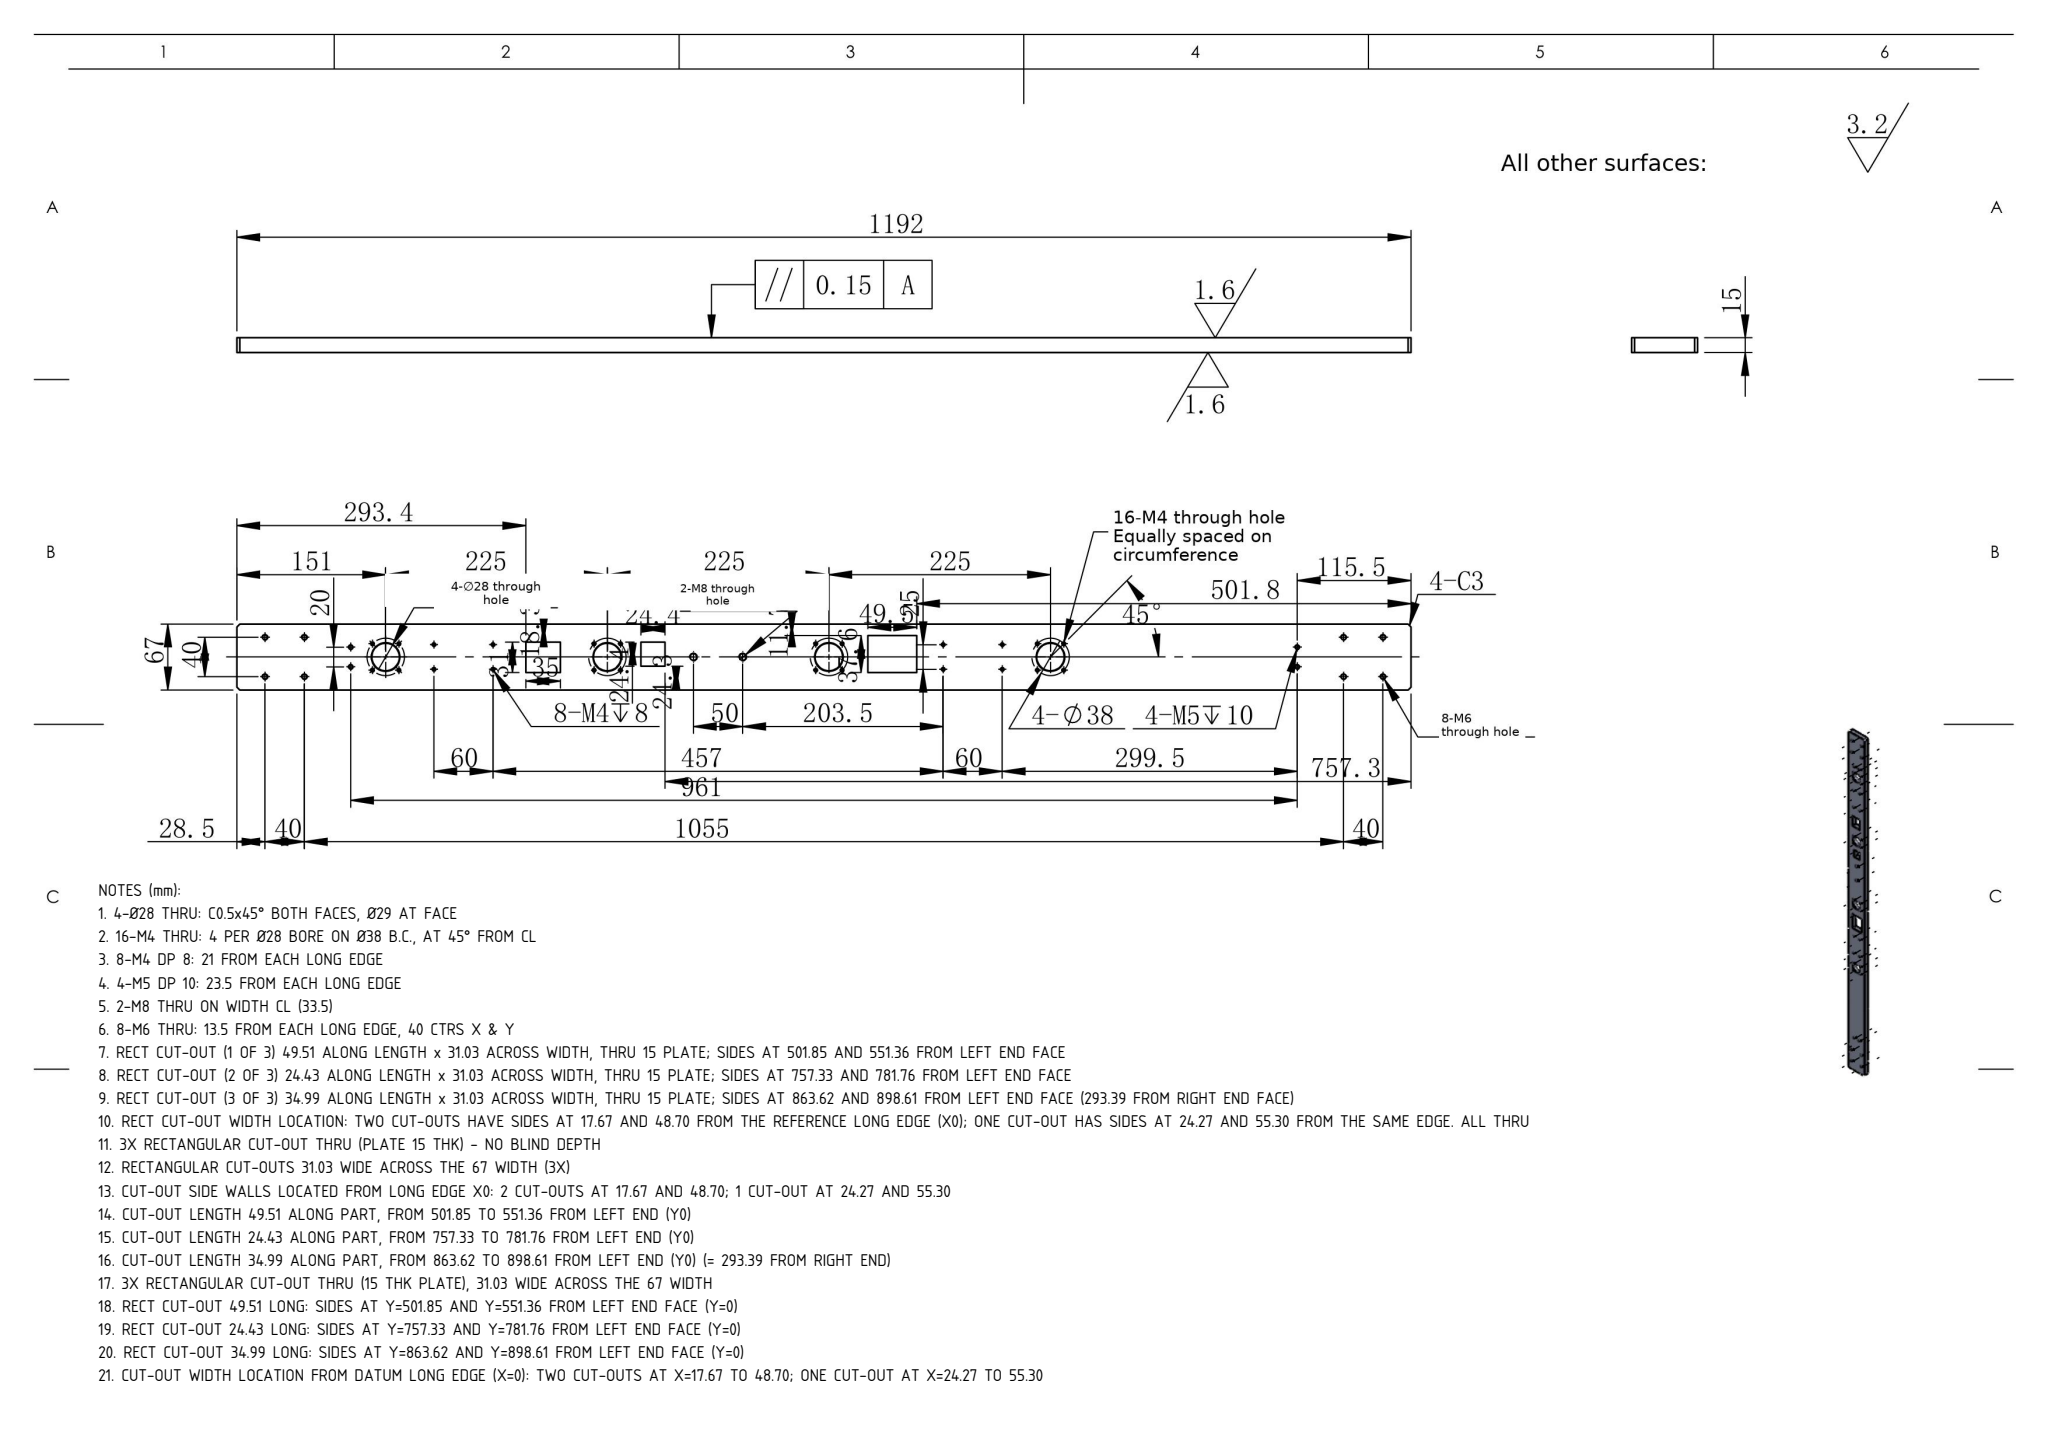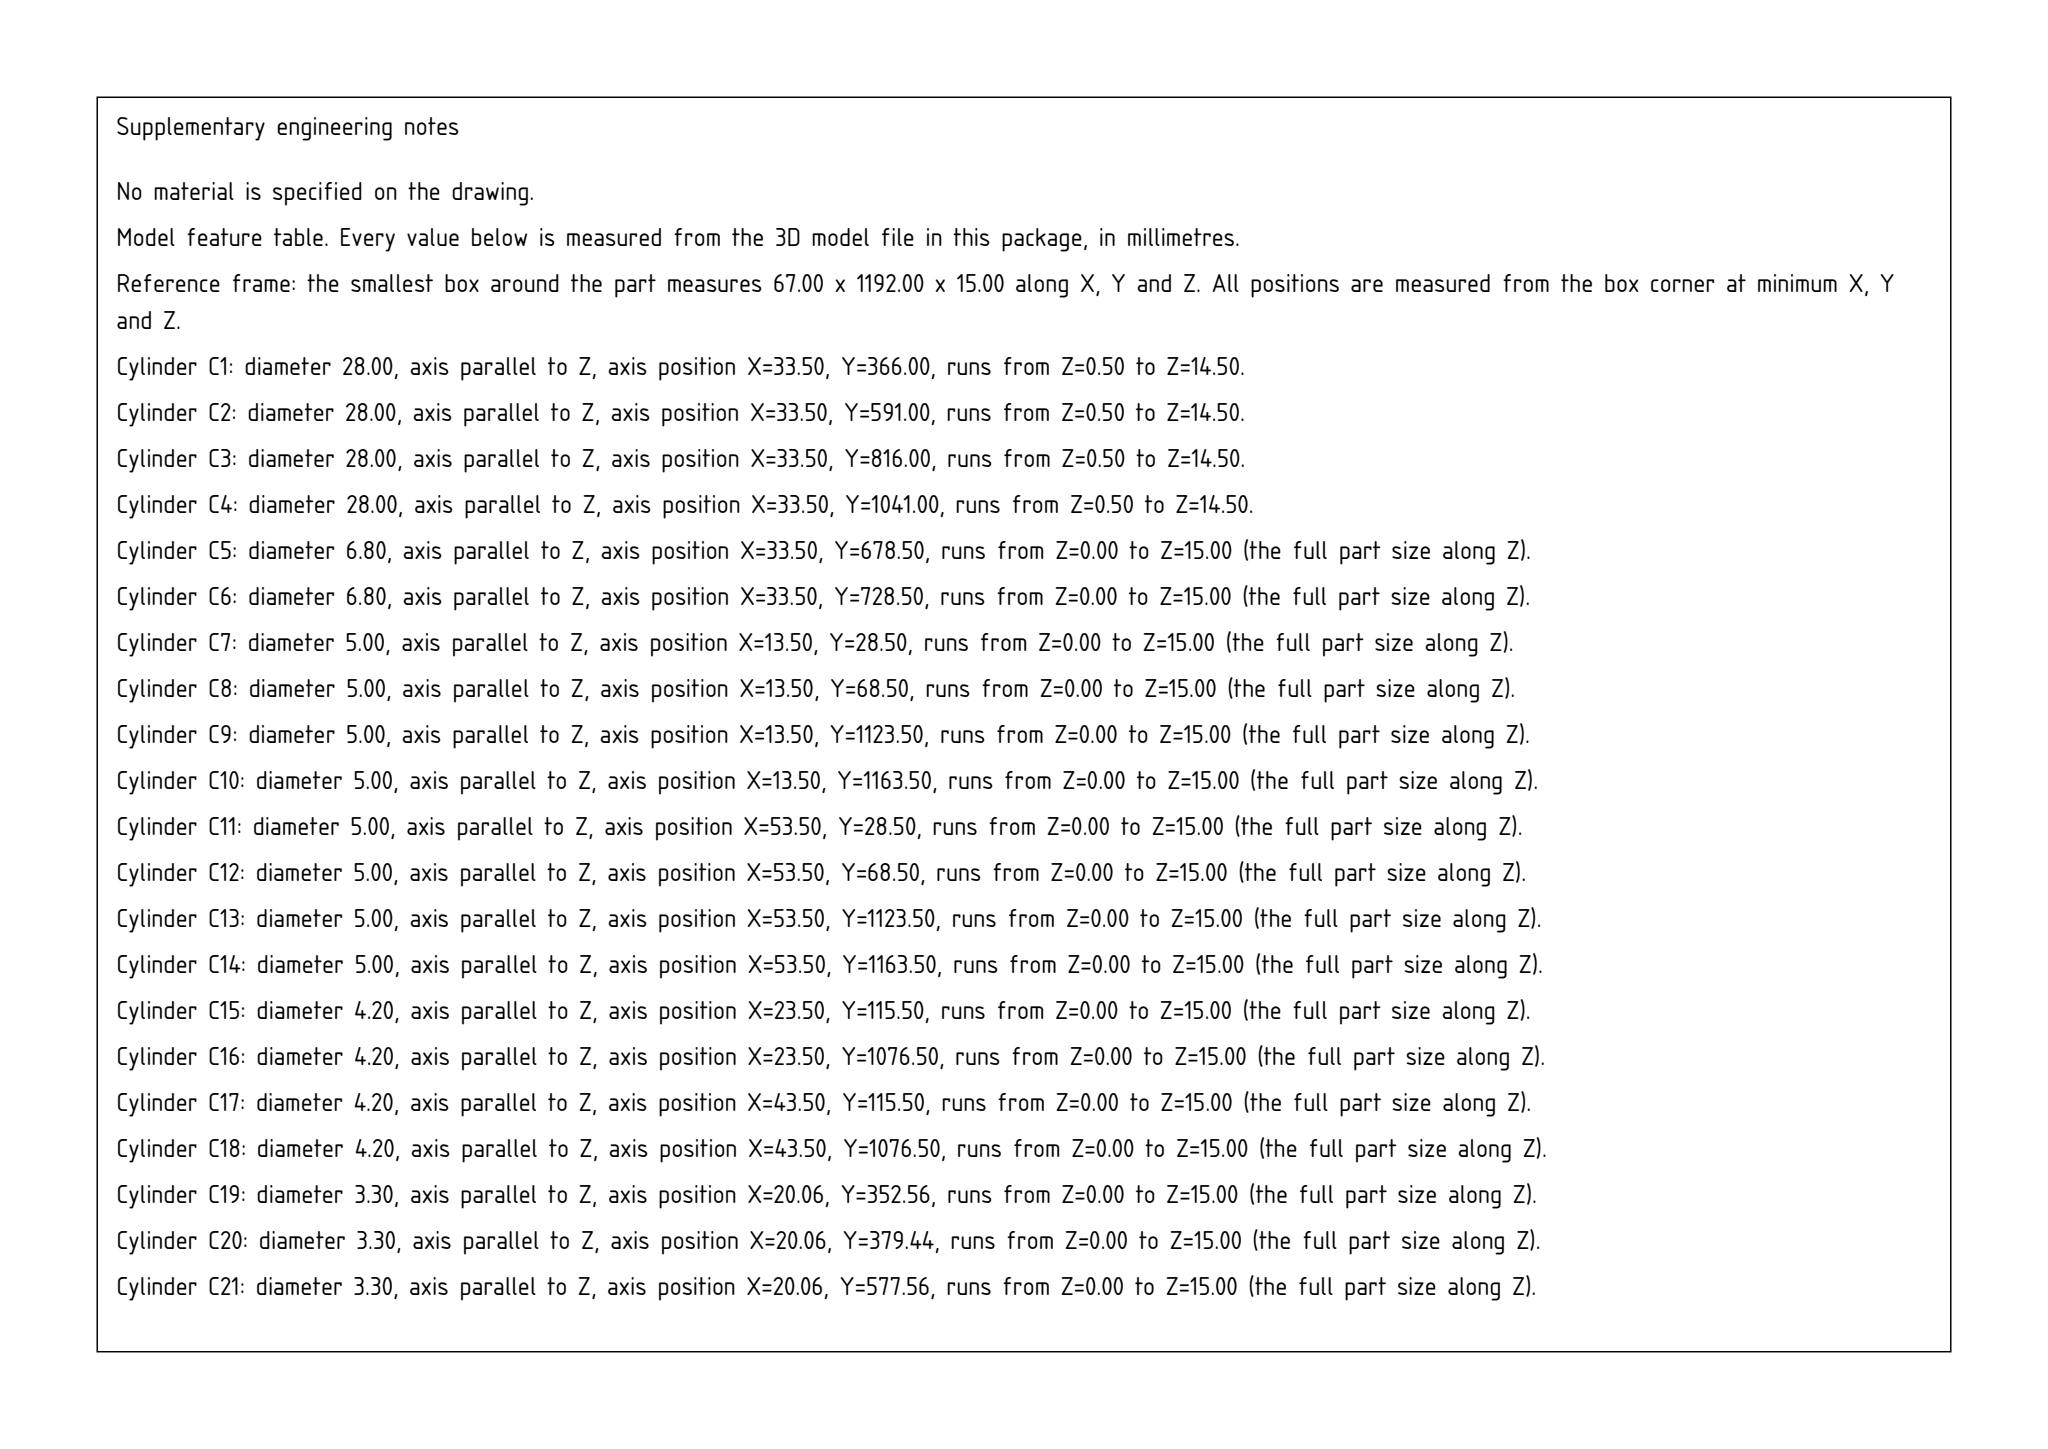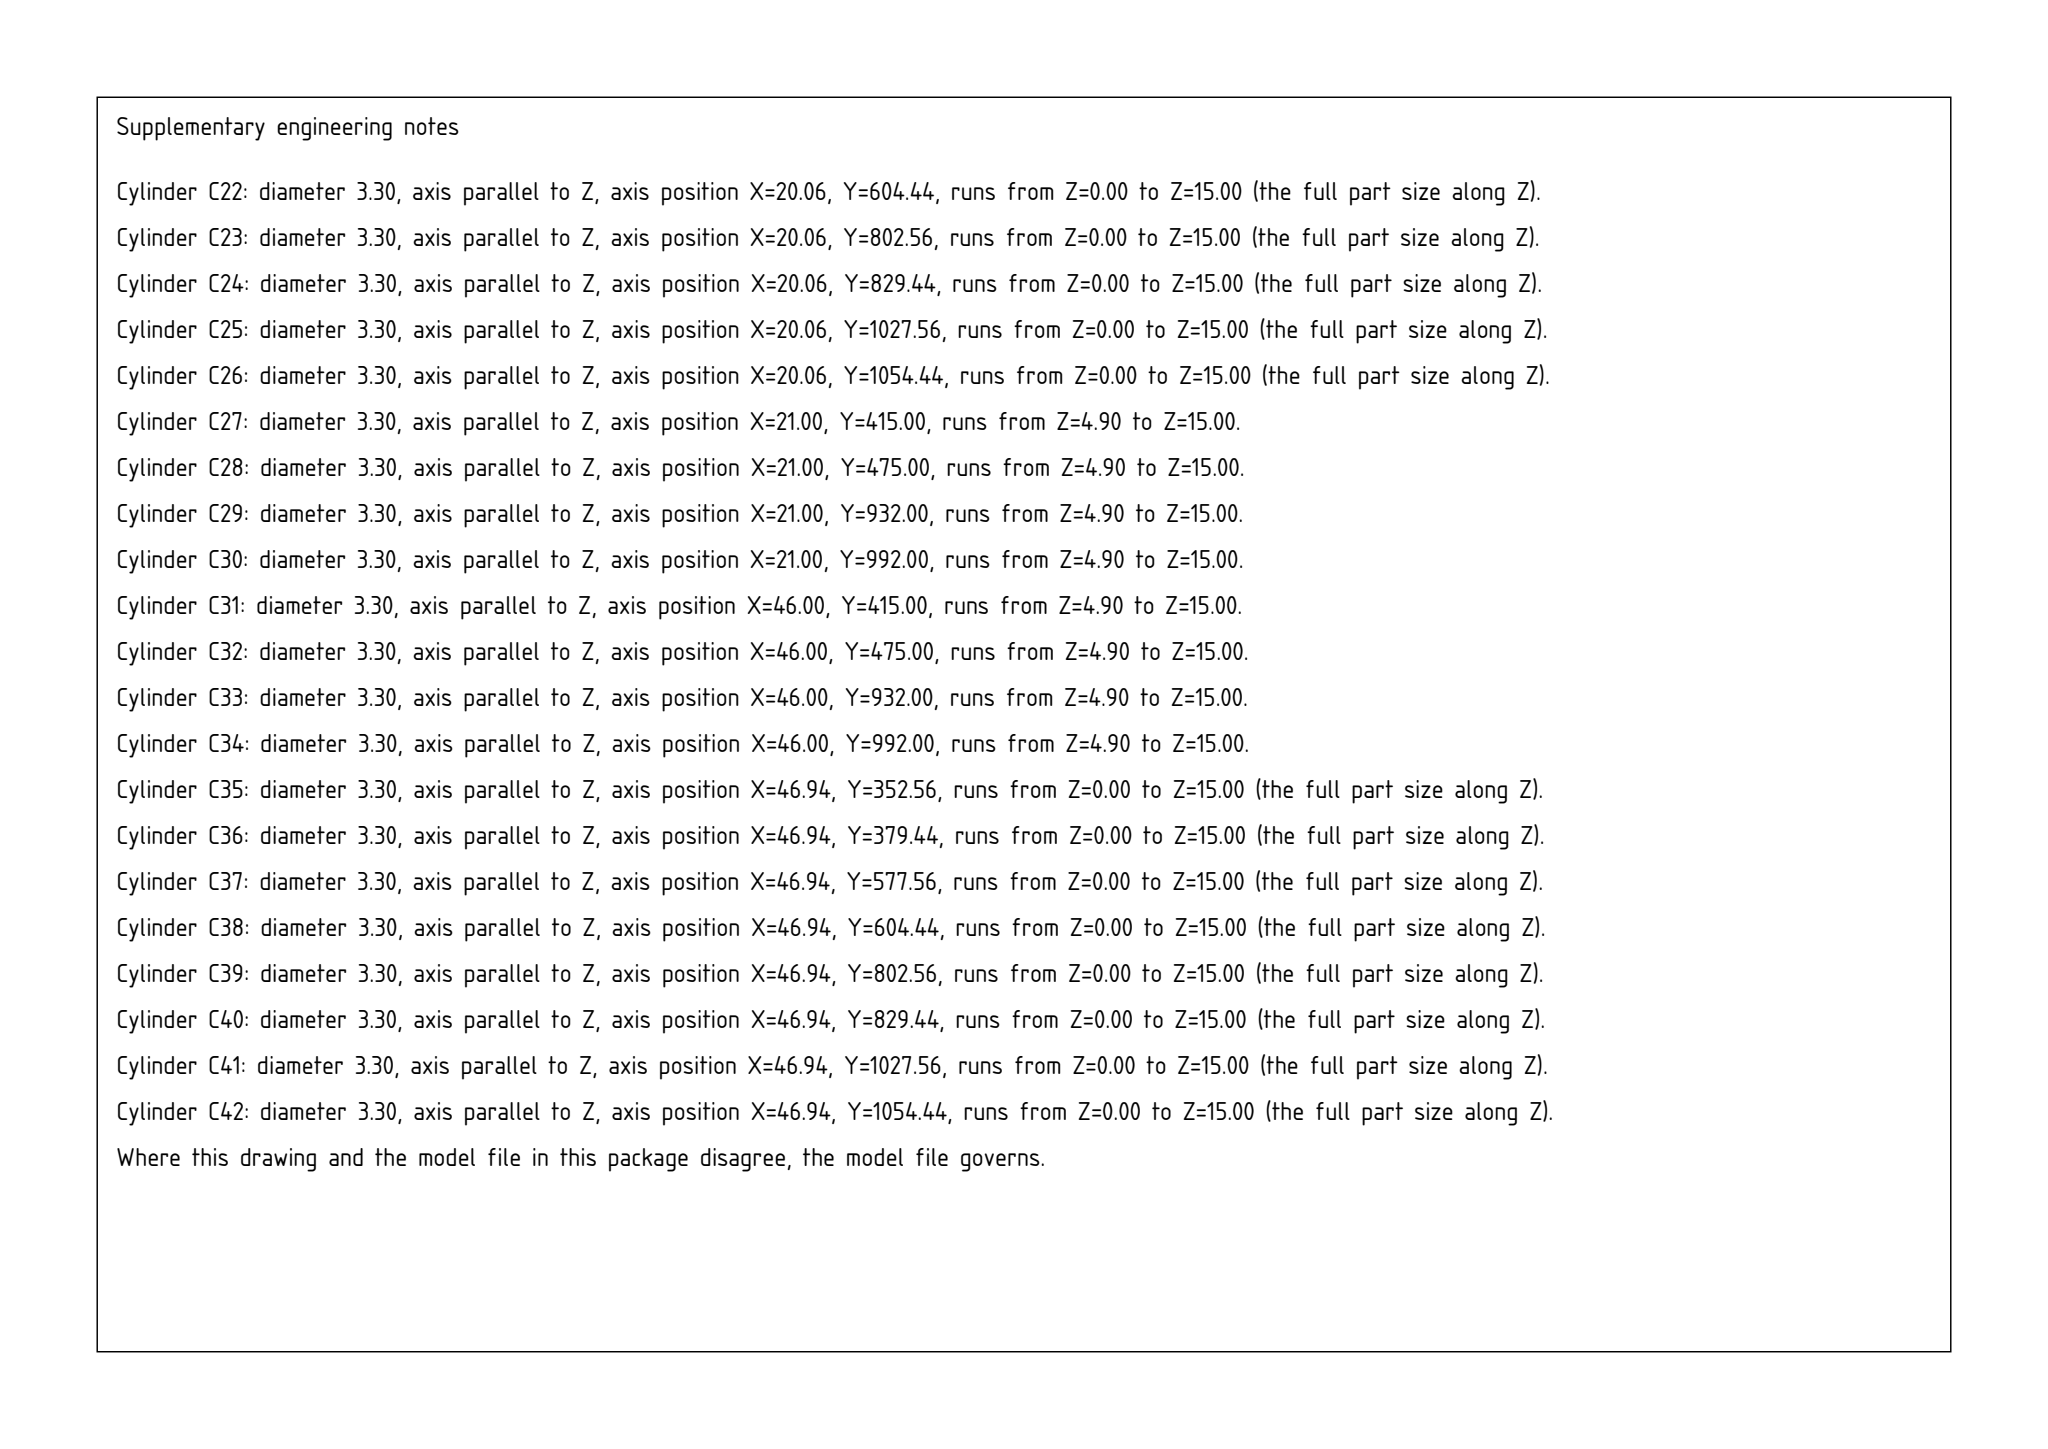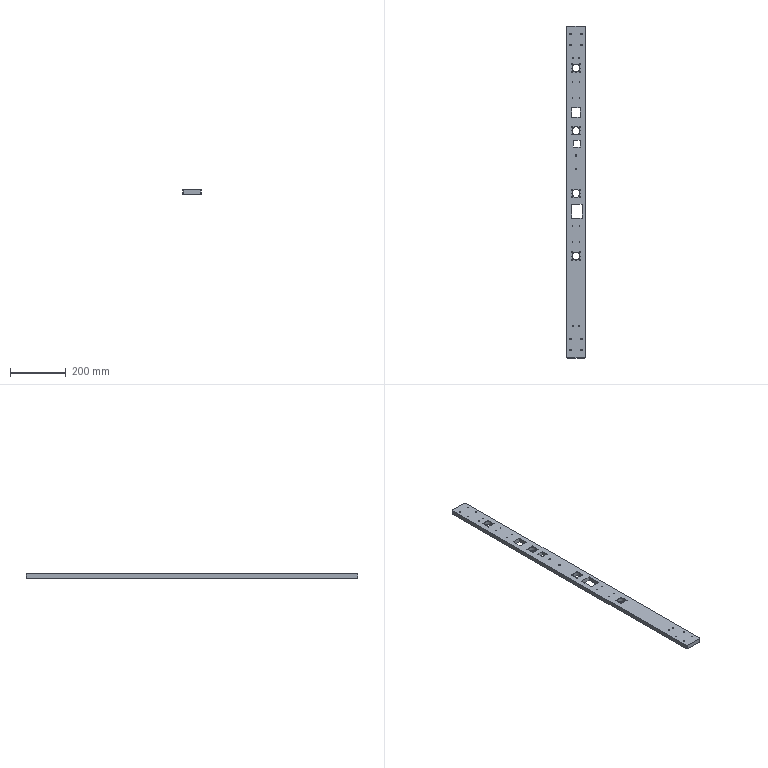Part | SolidWorks | mm | 1 solid | 138 faces | box 67 x 1192 x 15 mm | volume 1100432 mm3 | cylinder 84 | cone 32 | plane 22 | commonest cylinder face diameters 3.3 x48 5 x16 4.2 x8 28 x8 6.8 x4
Drawing notes:
4-Ø28 THRU: C0.5x45° BOTH FACES, Ø29 AT FACE | from the solid: Ø28 cyl L14.0 in 15 thk plate; 90° cones ref dia 28.0 (8) and 29.0 (8)
16-M4 THRU: 4 PER Ø28 BORE ON Ø38 B.C., AT 45° FROM CL | from the solid: Ø3.3 thru at x=20.06/46.94, y=352.56/379.44 etc = ±13.44,±13.44 from bore ctrs (33.5, 366/591/816/1041) -> R19 at 45°
8-M4 DP 8: 21 FROM EACH LONG EDGE | from the solid: Ø3.3 L10.1 at x=21 & 46 (67-46=21)
4-M5 DP 10: 23.5 FROM EACH LONG EDGE | from the solid: Ø4.2 at x=23.5 & 43.5 (67-43.5=23.5)
2-M8 THRU ON WIDTH CL (33.5) | from the solid: Ø6.8 thru at x=33.5 = 67/2 width CL, y=678.5 & 728.5
8-M6 THRU: 13.5 FROM EACH LONG EDGE, 40 CTRS X & Y | from the solid: Ø5.0 thru at x=13.5 & 53.5, y=28.5/68.5 and 1123.5/1163.5; bbox 67 x 1192
RECT CUT-OUT (1 OF 3) 49.51 ALONG LENGTH x 31.03 ACROSS WIDTH, THRU 15 PLATE; SIDES AT 501.85 AND 551.36 FROM LEFT END FACE | from the solid: axis_planes y=501.85 and y=551.36 (49.51 apart); x plane pair spacing 31.03; z planes only 0.0 and 15.0 (no blind floor)
RECT CUT-OUT (2 OF 3) 24.43 ALONG LENGTH x 31.03 ACROSS WIDTH, THRU 15 PLATE; SIDES AT 757.33 AND 781.76 FROM LEFT END FACE | from the solid: axis_planes y=757.33 and y=781.76 (24.43 apart); x plane pair spacing 31.03; z planes only 0.0 and 15.0
RECT CUT-OUT (3 OF 3) 34.99 ALONG LENGTH x 31.03 ACROSS WIDTH, THRU 15 PLATE; SIDES AT 863.62 AND 898.61 FROM LEFT END FACE (293.39 FROM RIGHT END FACE) | from the solid: axis_planes y=863.62 and y=898.61 (34.99 apart); bbox y=1192.0 gives 293.39 to right end; x plane pair spacing 31.03; z planes only 0.0 and 15.0
RECT CUT-OUT WIDTH LOCATION: TWO CUT-OUTS HAVE SIDES AT 17.67 AND 48.70 FROM THE REFERENCE LONG EDGE (X0); ONE CUT-OUT HAS SIDES AT 24.27 AND 55.30 FROM THE SAME EDGE. ALL THRU | from the solid: axis_planes x=17.67 (count 2), x=48.70 (count 2), x=24.27 (count 1), x=55.30 (count 1); bbox x=67.0
3X RECTANGULAR CUT-OUT THRU (PLATE 15 THK) - NO BLIND DEPTH | from the solid: axis_planes z 0.0 and z 15.0 are the only z faces; bbox_xyz z = 15.0, so cut-out walls run full thickness
RECTANGULAR CUT-OUTS 31.03 WIDE ACROSS THE 67 WIDTH (3X) | from the solid: axis_planes x 48.70 - x 17.67 = 31.03 and x 55.30 - x 24.27 = 31.03
CUT-OUT SIDE WALLS LOCATED FROM LONG EDGE X0: 2 CUT-OUTS AT 17.67 AND 48.70; 1 CUT-OUT AT 24.27 AND 55.30 | from the solid: axis_planes x 17.67 count 2, x 48.70 count 2, x 24.27 count 1, x 55.30 count 1
CUT-OUT LENGTH 49.51 ALONG PART, FROM 501.85 TO 551.36 FROM LEFT END (Y0) | from the solid: axis_planes y 501.85 and y 551.36
CUT-OUT LENGTH 24.43 ALONG PART, FROM 757.33 TO 781.76 FROM LEFT END (Y0) | from the solid: axis_planes y 757.33 and y 781.76
CUT-OUT LENGTH 34.99 ALONG PART, FROM 863.62 TO 898.61 FROM LEFT END (Y0) (= 293.39 FROM RIGHT END) | from the solid: axis_planes y 863.62 and y 898.61; bbox y = 1192.0
3X RECTANGULAR CUT-OUT THRU (15 THK PLATE), 31.03 WIDE ACROSS THE 67 WIDTH | from the solid: axis_planes x 17.67 & 48.70 (and 24.27 & 55.30) give 31.03 opening; z planes 0.0 and 15.0 = through thickness
RECT CUT-OUT 49.51 LONG: SIDES AT Y=501.85 AND Y=551.36 FROM LEFT END FACE (Y=0) | from the solid: axis_planes y 501.85 and y 551.36
RECT CUT-OUT 24.43 LONG: SIDES AT Y=757.33 AND Y=781.76 FROM LEFT END FACE (Y=0) | from the solid: axis_planes y 757.33 and y 781.76
RECT CUT-OUT 34.99 LONG: SIDES AT Y=863.62 AND Y=898.61 FROM LEFT END FACE (Y=0) | from the solid: axis_planes y 863.62 and y 898.61
CUT-OUT WIDTH LOCATION FROM DATUM LONG EDGE (X=0): TWO CUT-OUTS AT X=17.67 TO 48.70; ONE CUT-OUT AT X=24.27 TO 55.30 | from the solid: axis_planes x 17.67 (count 2), 48.70 (count 2), 24.27 (count 1), 55.30 (count 1)
build123d program:
from build123d import *

# Parameters (mm, degrees)
SKETCH1_W             = 67
SKETCH1_H             = 1175
BOSS_EXTRUDE1_DEPTH   = 15
M6_TAPPED_HOLE1_D     = 5
SKETCH4_R             = 14
CUT_EXTRUDE1_DEPTH    = 1178.004
M8_TAPPED_HOLE1_D     = 6.8
M8_TAPPED_HOLE1_DEPTH = 19.75
M8_TAPPED_HOLE1_TIP   = 2.043
M4_TAPPED_HOLE1_D     = 3.3
CIRPATTERN1_COUNT     = 4
LPATTERN1_COUNT       = 4
LPATTERN1_PITCH       = 225
LPATTERN1_COPY_1_D    = 3.3
LPATTERN1_COPY_2_D    = 3.3
LPATTERN1_COPY_3_D    = 3.3
LPATTERN1_COPY_4_D    = 3.3
LPATTERN1_COPY_5_D    = 3.3
LPATTERN1_COPY_6_D    = 3.3
LPATTERN1_COPY_7_D    = 3.3
LPATTERN1_COPY_8_D    = 3.3
LPATTERN1_COPY_9_D    = 3.3
CHAMFER2_SIZE         = 0.5
M4_TAPPED_HOLE2_D     = 3.3
M4_TAPPED_HOLE2_DEPTH = 10.1
M4_TAPPED_HOLE2_TIP   = 0.9914
SKETCH11_W            = 67
SKETCH11_H            = 15
BOSS_EXTRUDE2_DEPTH   = 8.5
SKETCH12_W            = 67
SKETCH12_H            = 15
BOSS_EXTRUDE3_DEPTH   = 8.5
CHAMFER3_SIZE         = 3
M5_TAPPED_HOLE1_D     = 4.2
SKETCH15_W            = 31.028
SKETCH15_H            = 34.989
SKETCH15_W_2          = 24.426
SKETCH15_H_2          = 24.426
SKETCH15_W_3          = 37.629
SKETCH15_H_3          = 49.512
CUT_EXTRUDE2_DEPTH    = 104


with BuildPart() as part:
    # Sketch1 → Boss-Extrude1 (new body)
    with BuildSketch(Plane.XY):
        with Locations((33.5, 587.5)):
            Rectangle(SKETCH1_W, SKETCH1_H)
    extrude(amount=BOSS_EXTRUDE1_DEPTH)

    # M6 Tapped Hole1 (through all)
    with Locations(Plane.XY.offset(15)):
        with Locations((13.5, 1155), (53.5, 1155), (53.5, 1115), (13.5, 1115), (13.5, 60), (53.5, 60), (53.5, 20), (13.5, 20)):
            Hole(M6_TAPPED_HOLE1_D / 2)

    # Sketch4 → Cut-Extrude1 (cut, through all)
    with BuildSketch(Plane.XY.offset(15)):
        with Locations((33.5, 1032.5)):
            Circle(SKETCH4_R)
        with Locations(Location((33.5, 357.5, 0), (0, 0, 180))):
            Circle(SKETCH4_R)
        with Locations((33.5, 807.5)):
            Circle(SKETCH4_R)
        with Locations(Location((33.5, 582.5, 0), (0, 0, 180))):
            Circle(SKETCH4_R)
    extrude(amount=-CUT_EXTRUDE1_DEPTH, mode=Mode.SUBTRACT)

    # M8 Tapped Hole1
    with Locations(Plane.XY.offset(15)):
        with Locations((33.5, 720), (33.5, 670)):
            Hole(M8_TAPPED_HOLE1_D / 2, depth=M8_TAPPED_HOLE1_DEPTH)
            with Locations((0, 0, -(M8_TAPPED_HOLE1_DEPTH + M8_TAPPED_HOLE1_TIP / 2))):  # 118° drill point
                Cone(0, M8_TAPPED_HOLE1_D / 2, M8_TAPPED_HOLE1_TIP, mode=Mode.SUBTRACT)

    # M4 Tapped Hole1 (through all)
    with Locations(Plane.XY.offset(15)):
        with Locations((46.935, 1045.935)):
            m4_tapped_hole1 = Hole(M4_TAPPED_HOLE1_D / 2)

    # CirPattern1: M4 Tapped Hole1 ×4 about axis
    cirpattern1_axis = Axis((33.5, 1032.5, 0), (0, 0, 1))
    for i in range(1, CIRPATTERN1_COUNT):
        add(m4_tapped_hole1.rotate(cirpattern1_axis, i * 360 / CIRPATTERN1_COUNT), mode=Mode.SUBTRACT)

    # LPattern1: M4 Tapped Hole1 ×4
    with Locations(*[(0, -i * LPATTERN1_PITCH, 0) for i in range(1, LPATTERN1_COUNT)]):
        add(m4_tapped_hole1, mode=Mode.SUBTRACT)

    # LPattern1 copy 1 (through all)
    with Locations(Plane(origin=(1066, 774, 15), x_dir=(0, 1, 0), z_dir=(0, 0, 1))):
        with Locations((46.935, 1045.935)):
            Hole(LPATTERN1_COPY_1_D / 2)

    # LPattern1 copy 2 (through all)
    with Locations(Plane(origin=(1066, 549, 15), x_dir=(0, 1, 0), z_dir=(0, 0, 1))):
        with Locations((46.935, 1045.935)):
            Hole(LPATTERN1_COPY_2_D / 2)

    # LPattern1 copy 3 (through all)
    with Locations(Plane(origin=(1066, 324, 15), x_dir=(0, 1, 0), z_dir=(0, 0, 1))):
        with Locations((46.935, 1045.935)):
            Hole(LPATTERN1_COPY_3_D / 2)

    # LPattern1 copy 4 (through all)
    with Locations(Plane(origin=(67, 1840, 15), x_dir=(-1, 0, 0), z_dir=(0, 0, 1))):
        with Locations((46.935, 1045.935)):
            Hole(LPATTERN1_COPY_4_D / 2)

    # LPattern1 copy 5 (through all)
    with Locations(Plane(origin=(67, 1615, 15), x_dir=(-1, 0, 0), z_dir=(0, 0, 1))):
        with Locations((46.935, 1045.935)):
            Hole(LPATTERN1_COPY_5_D / 2)

    # LPattern1 copy 6 (through all)
    with Locations(Plane(origin=(67, 1390, 15), x_dir=(-1, 0, 0), z_dir=(0, 0, 1))):
        with Locations((46.935, 1045.935)):
            Hole(LPATTERN1_COPY_6_D / 2)

    # LPattern1 copy 7 (through all)
    with Locations(Plane(origin=(-999, 841, 15), x_dir=(0, -1, 0), z_dir=(0, 0, 1))):
        with Locations((46.935, 1045.935)):
            Hole(LPATTERN1_COPY_7_D / 2)

    # LPattern1 copy 8 (through all)
    with Locations(Plane(origin=(-999, 616, 15), x_dir=(0, -1, 0), z_dir=(0, 0, 1))):
        with Locations((46.935, 1045.935)):
            Hole(LPATTERN1_COPY_8_D / 2)

    # LPattern1 copy 9 (through all)
    with Locations(Plane(origin=(-999, 391, 15), x_dir=(0, -1, 0), z_dir=(0, 0, 1))):
        with Locations((46.935, 1045.935)):
            Hole(LPATTERN1_COPY_9_D / 2)

    # Chamfer2
    chamfer2_edges = [part.edges().sort_by_distance(p)[0] for p in [
        (19.5, 1032.5, 0),
        (19.5, 1032.5, 15),
        (47.5, 357.5, 0),
        (47.5, 357.5, 15),
        (19.5, 807.5, 0),
        (19.5, 807.5, 15),
        (47.5, 582.5, 0),
        (47.5, 582.5, 15),
    ]]
    chamfer(chamfer2_edges, length=CHAMFER2_SIZE)

    # M4 Tapped Hole2
    with Locations(Plane.XY.offset(15)):
        with Locations((46, 983.5), (21, 983.5), (21, 923.5), (46, 923.5), (46, 466.5), (21, 466.5), (21, 406.5), (46, 406.5)):
            Hole(M4_TAPPED_HOLE2_D / 2, depth=M4_TAPPED_HOLE2_DEPTH)
            with Locations((0, 0, -(M4_TAPPED_HOLE2_DEPTH + M4_TAPPED_HOLE2_TIP / 2))):  # 118° drill point
                Cone(0, M4_TAPPED_HOLE2_D / 2, M4_TAPPED_HOLE2_TIP, mode=Mode.SUBTRACT)

    # Sketch11 → Boss-Extrude2 (add)
    with BuildSketch(Plane(origin=(0, 1175, 0), x_dir=(1, 0, 0), z_dir=(0, 1, 0))):
        with Locations((33.5, -7.5)):
            Rectangle(SKETCH11_W, SKETCH11_H)
    extrude(amount=BOSS_EXTRUDE2_DEPTH)

    # Sketch12 → Boss-Extrude3 (add)
    with BuildSketch(Plane.XZ):
        with Locations((33.5, 7.5)):
            Rectangle(SKETCH12_W, SKETCH12_H)
    extrude(amount=BOSS_EXTRUDE3_DEPTH)

    # Chamfer3
    chamfer3_edges = [part.edges().sort_by_distance(p)[0] for p in [
        (0, 1183.5, 7.5),
        (67, 1183.5, 7.5),
        (0, -8.5, 7.5),
        (67, -8.5, 7.5),
    ]]
    chamfer(chamfer3_edges, length=CHAMFER3_SIZE)

    # M5 Tapped Hole1 (through all)
    with Locations(Plane.XY.offset(15)):
        with Locations((43.5, 1068), (23.5, 1068), (23.5, 107), (43.5, 107)):
            Hole(M5_TAPPED_HOLE1_D / 2)

    # Sketch15 → Cut-Extrude2 (cut)
    with BuildSketch(Plane.XY.offset(15)):
        with Locations((33.187, 872.613)):
            Rectangle(SKETCH15_W, SKETCH15_H)
        with Locations((36.488, 761.045)):
            Rectangle(SKETCH15_W_2, SKETCH15_H_2)
        with Locations((36.488, 518.104)):
            Rectangle(SKETCH15_W_3, SKETCH15_H_3)
    extrude(amount=-CUT_EXTRUDE2_DEPTH, mode=Mode.SUBTRACT)


solid = part.part